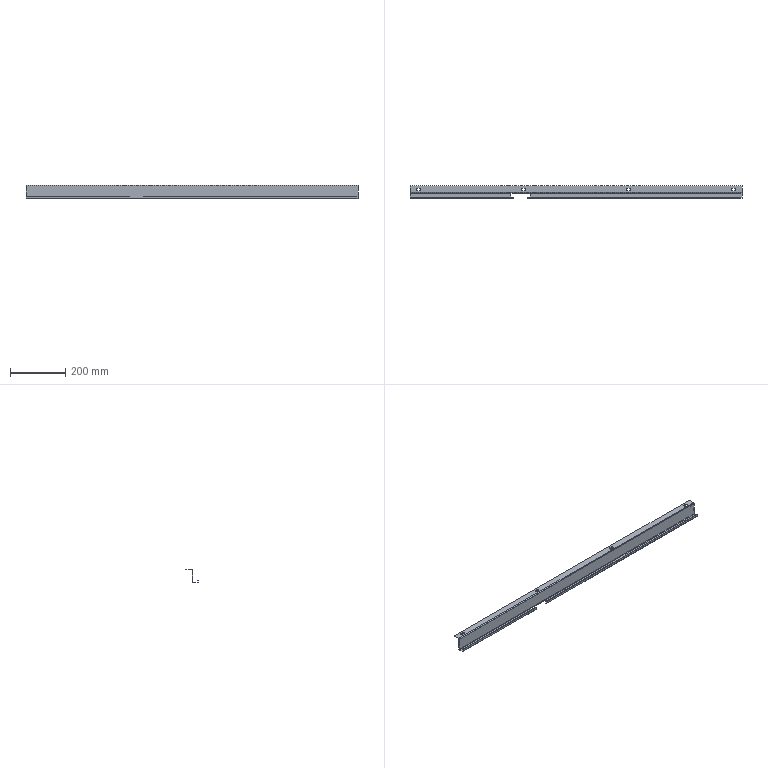Component | SolidWorks | BoxUpperBeam2-1 | 1 solid | 64 faces | volume 172560 mm3 | plane 48 | cylinder 16 | commonest cylinder face diameters 9 x8 3 x4 6 x4